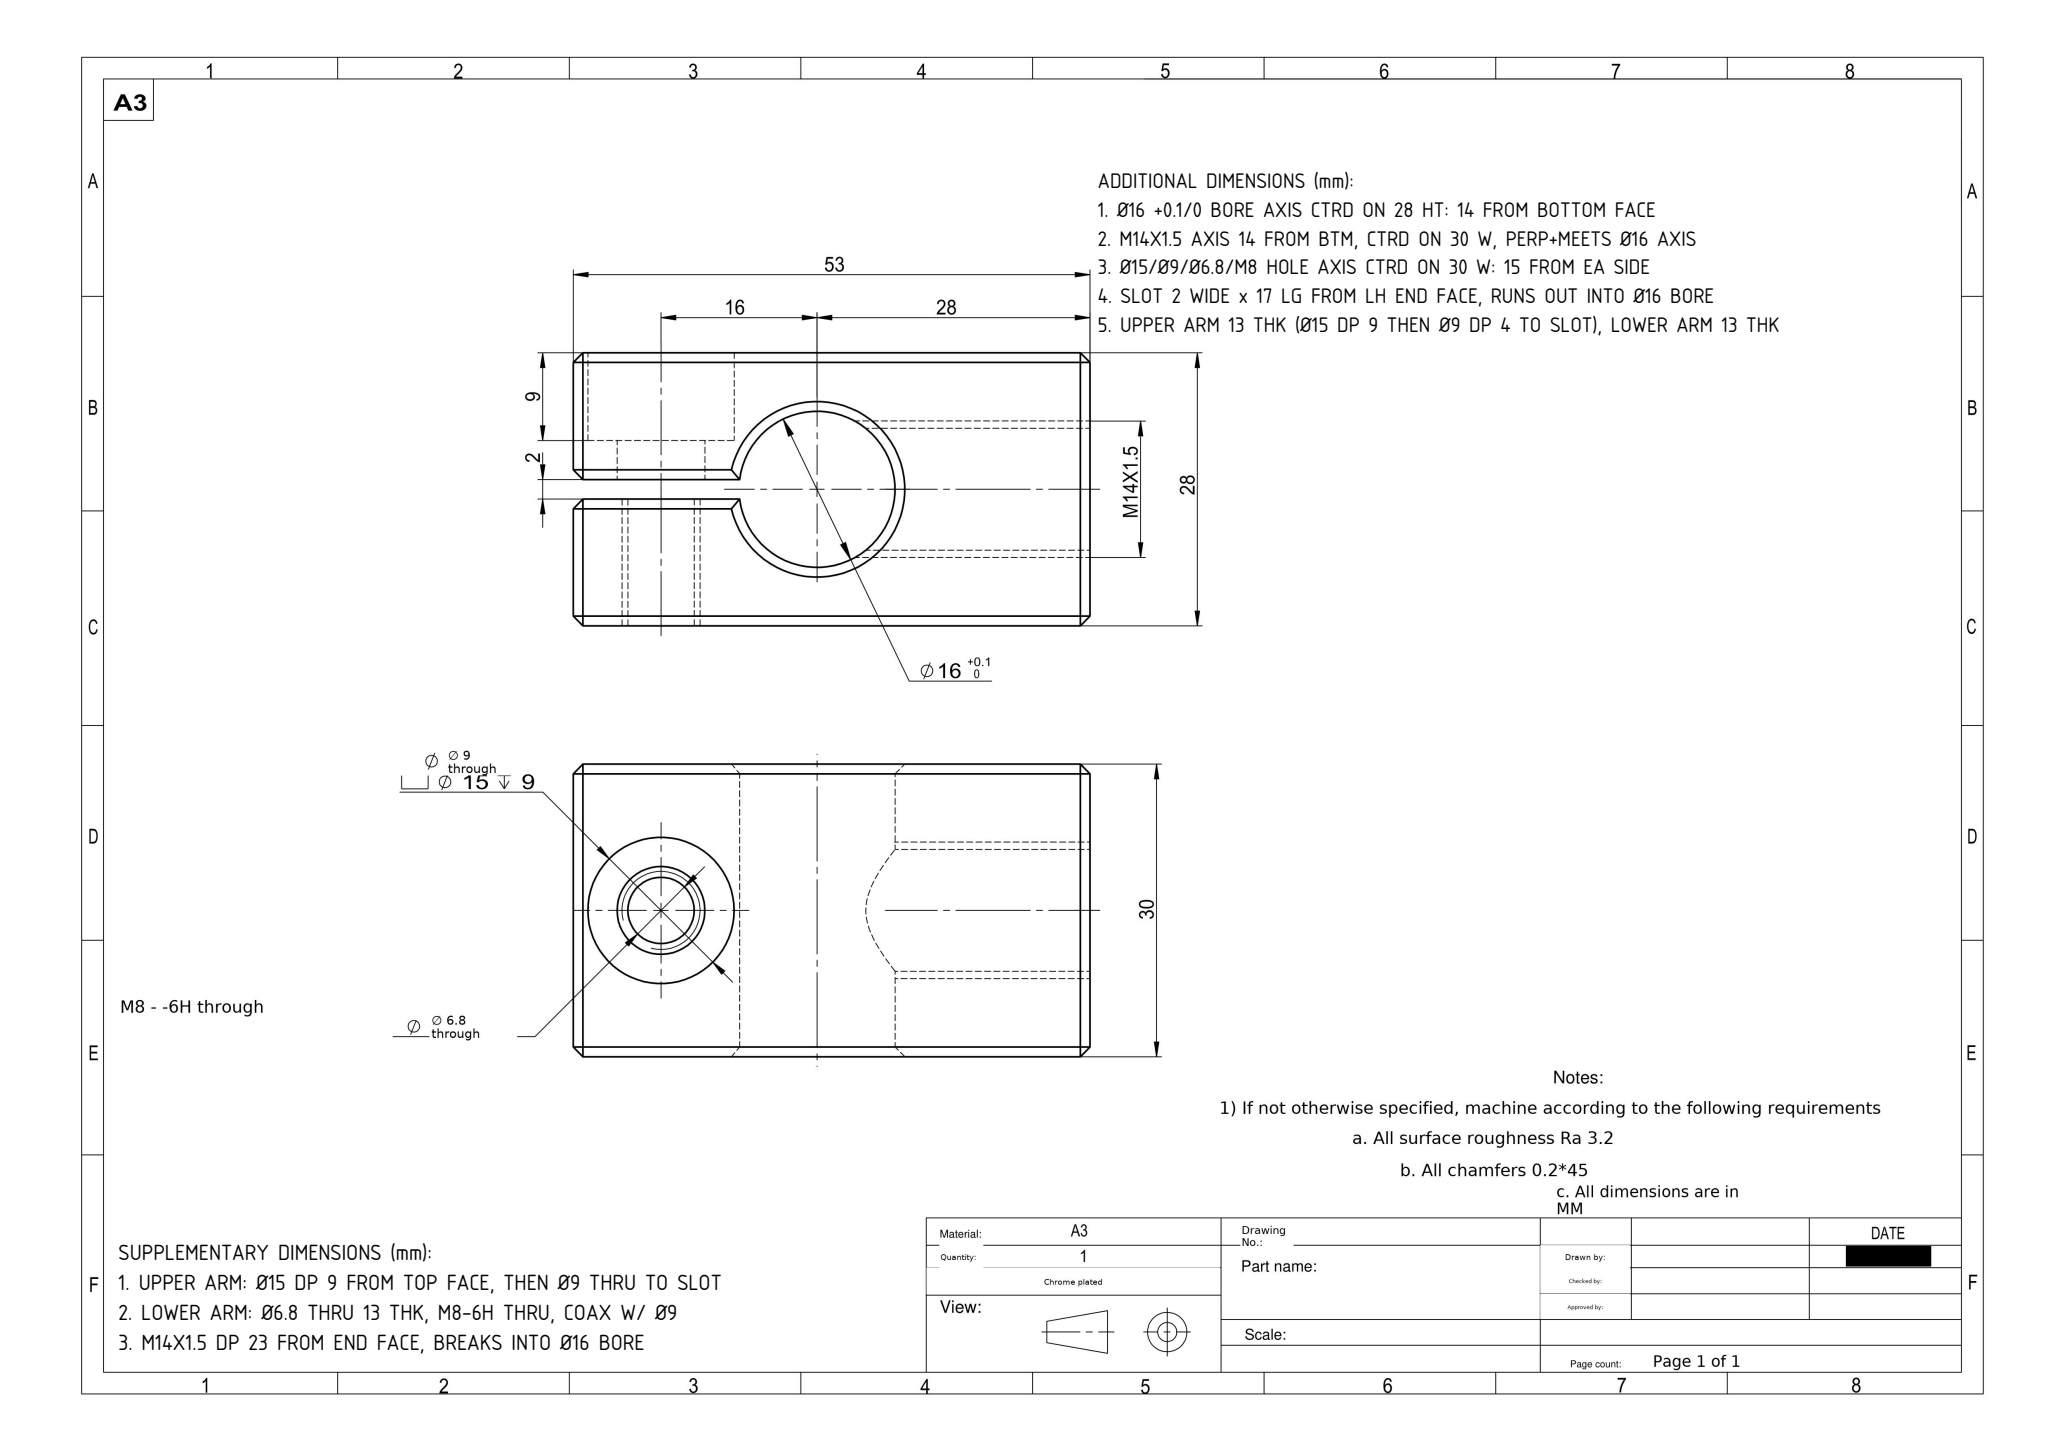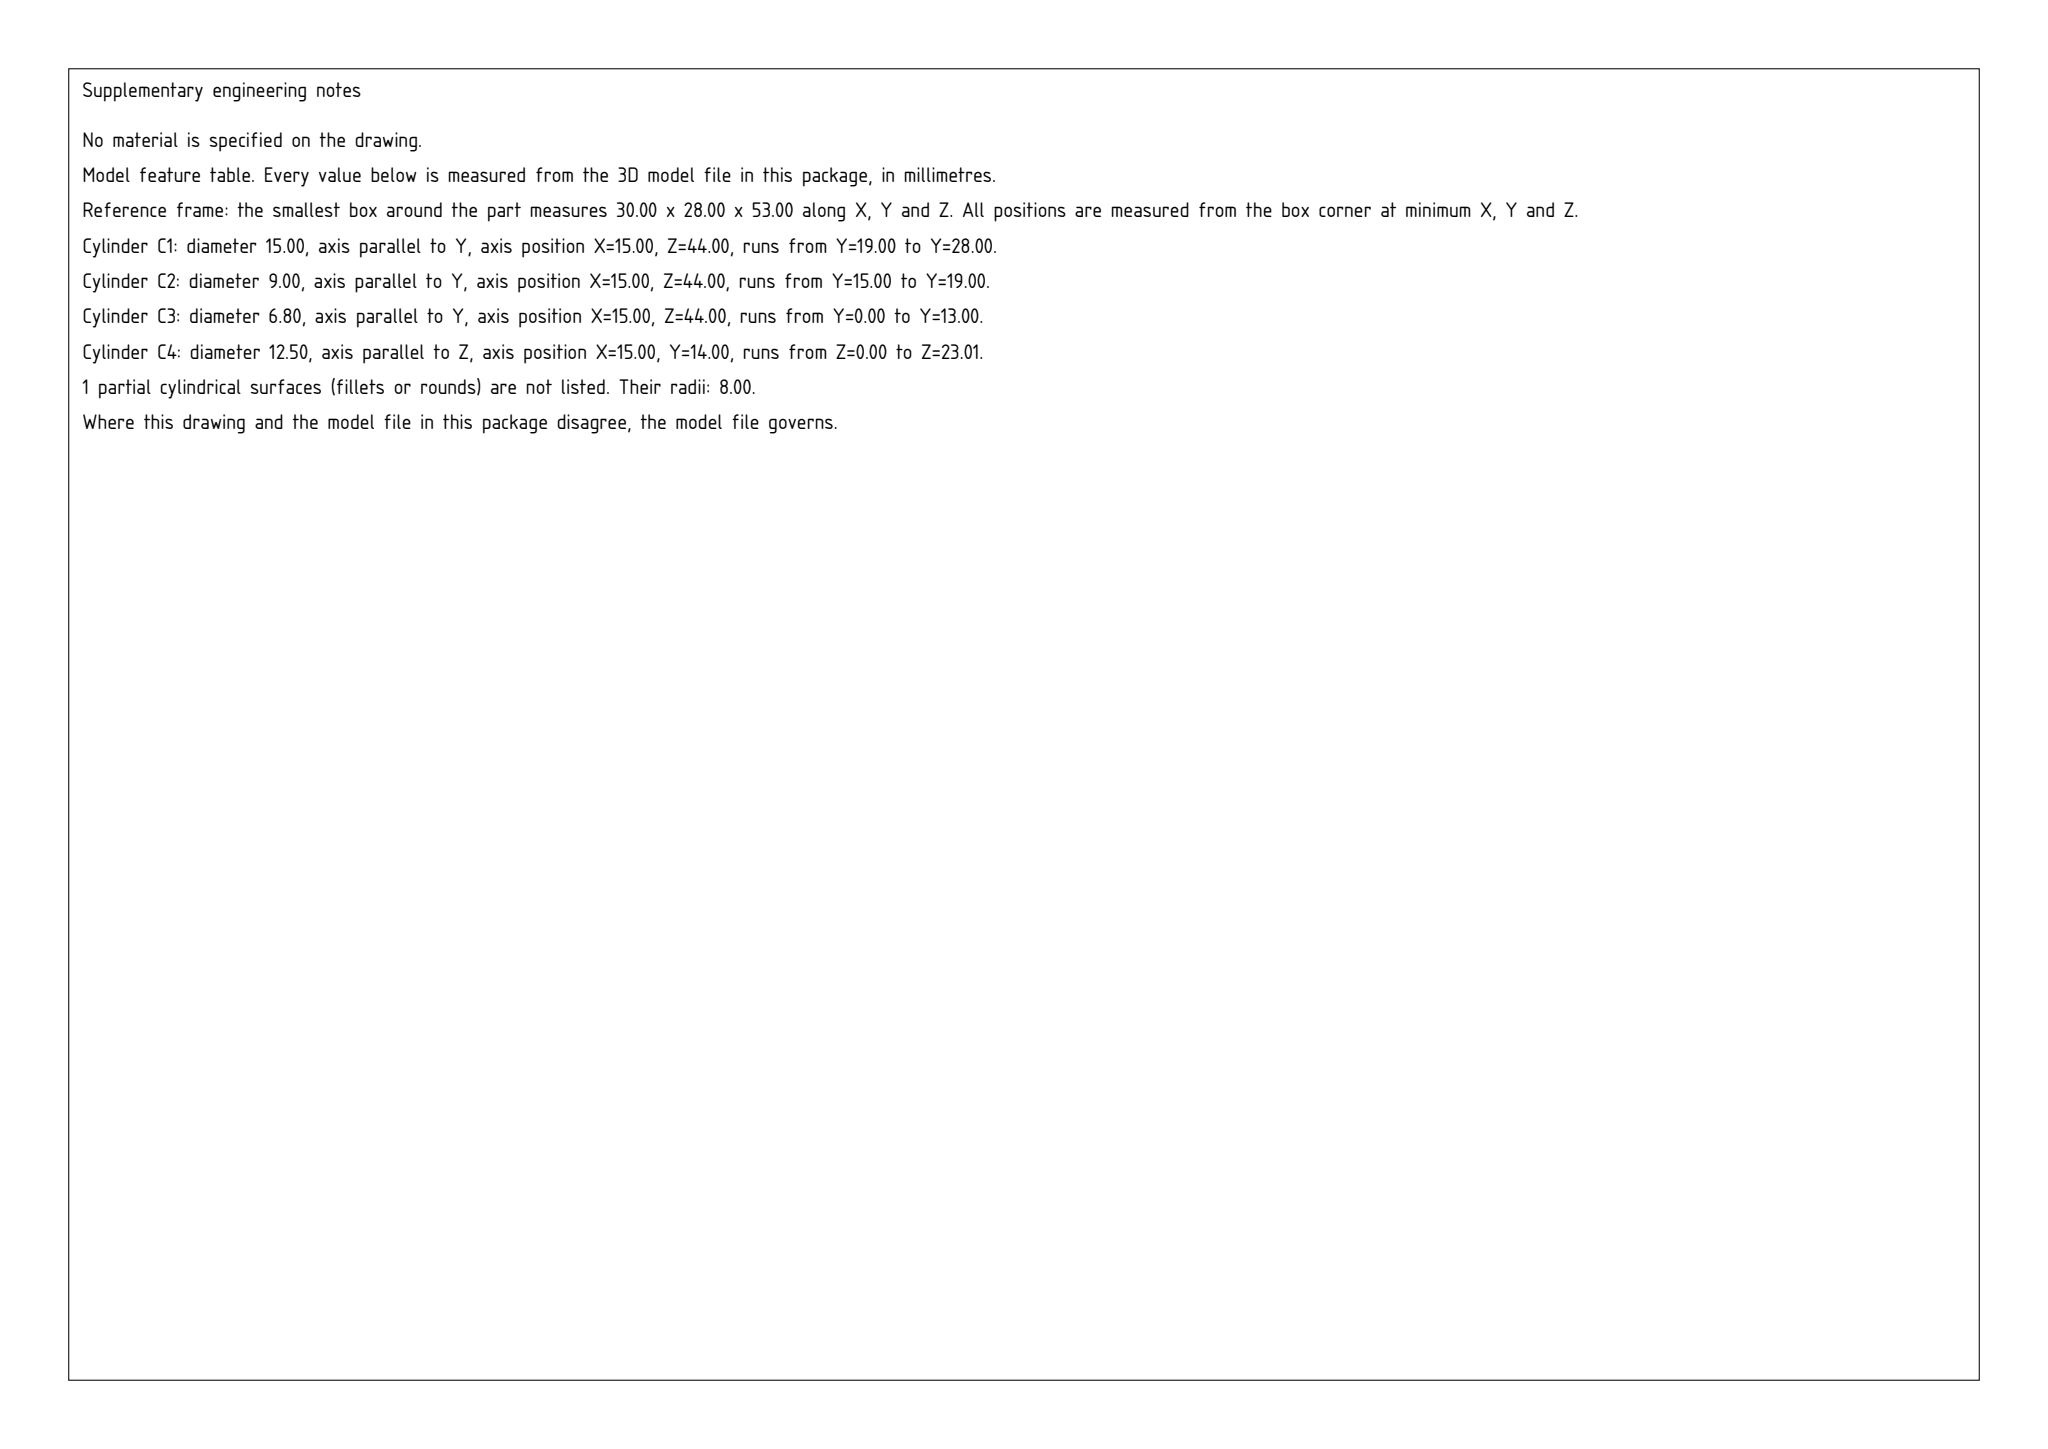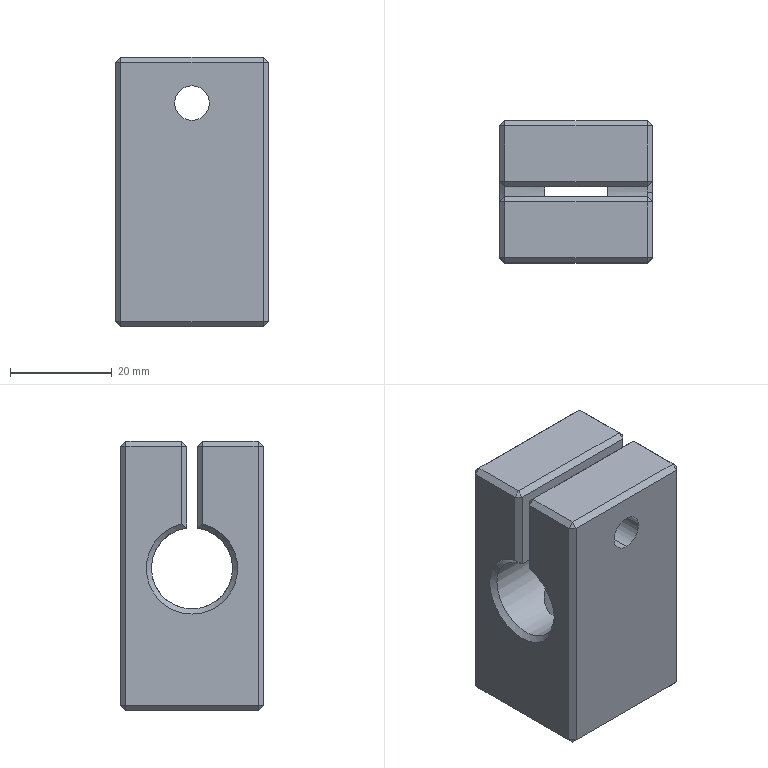Part | SolidWorks | mm | 1 solid | 54 faces | box 30 x 28 x 53 mm | volume 32288 mm3 | plane 42 | cylinder 9 | cone 3 | commonest cylinder face diameters 6.8 x2 15 x2 9 x2 12.5 x2 16 x1
build123d program:
from build123d import *

# Parameters (mm, degrees)
SKETCH1_W                                         = 53
SKETCH1_H                                         = 28
SKETCH1_R                                         = 8
BOSS_EXTRUDE1_DEPTH                               = 15
M14X1_5_TAPPED_HOLE1_REACH                        = 58.833
M14X1_5_TAPPED_HOLE1_BORE_R                       = 6.25
CUT_EXTRUDE1_DEPTH                                = 35.713
CUT_EXTRUDE1_DEPTH_BACK                           = 35.713
SKETCH2_W                                         = 25
SKETCH2_H                                         = 2
HOLE_SIZE_ACCORDING_TO_HEXAGON_SOCKET_D           = 9
HOLE_SIZE_ACCORDING_TO_HEXAGON_SOCKET_DEPTH       = 13
HOLE_SIZE_ACCORDING_TO_HEXAGON_SOCKET_CBORE_D     = 15
HOLE_SIZE_ACCORDING_TO_HEXAGON_SOCKET_CBORE_DEPTH = 9
M8_TAPPED_HOLE1_D                                 = 6.8
CHAMFER1_SIZE                                     = 1


with BuildPart() as part:
    # Sketch1 → Boss-Extrude1 (new, symmetric)
    with BuildSketch(Plane(origin=(0, 0, 0), x_dir=(0, 0, -1), z_dir=(1, 0, 0))):
        with Locations((1.5, 0)):
            Rectangle(SKETCH1_W, SKETCH1_H)
        Circle(SKETCH1_R, mode=Mode.SUBTRACT)
    extrude(amount=BOSS_EXTRUDE1_DEPTH, both=True)

    # M14x1.5 Tapped Hole1 bore → M14x1.5 Tapped Hole1 (cut, up to next)
    with BuildSketch(Plane(origin=(0, 0, -28), x_dir=(-1, 0, 0), z_dir=(0, 0, -1)), mode=Mode.PRIVATE) as m14x1_5_tapped_hole1_sk1:
        Circle(M14X1_5_TAPPED_HOLE1_BORE_R)
    m14x1_5_tapped_hole1_tool1 = extrude(m14x1_5_tapped_hole1_sk1.sketch, amount=-M14X1_5_TAPPED_HOLE1_REACH, mode=Mode.PRIVATE) & part.part
    add(m14x1_5_tapped_hole1_tool1.solids().sort_by_distance((0, 0, -28))[0], mode=Mode.SUBTRACT)

    # Sketch2 → Cut-Extrude1 (cut, two sides: drawn at the far end of the back side and taken through both)
    with BuildSketch(Plane(origin=(0, 0, 0), x_dir=(0, 0, -1), z_dir=(1, 0, 0)).offset(-CUT_EXTRUDE1_DEPTH_BACK)):
        with Locations((-12.5, 0)):
            Rectangle(SKETCH2_W, SKETCH2_H)
    extrude(amount=CUT_EXTRUDE1_DEPTH + CUT_EXTRUDE1_DEPTH_BACK, mode=Mode.SUBTRACT)

    # Hole Size _ according to_ Hexagon Socket
    with Locations(Plane(origin=(0, 14, 0), x_dir=(1, 0, 0), z_dir=(0, 1, 0))):
        with Locations((0, -16)):
            CounterBoreHole(HOLE_SIZE_ACCORDING_TO_HEXAGON_SOCKET_D / 2, HOLE_SIZE_ACCORDING_TO_HEXAGON_SOCKET_CBORE_D / 2, HOLE_SIZE_ACCORDING_TO_HEXAGON_SOCKET_CBORE_DEPTH, depth=HOLE_SIZE_ACCORDING_TO_HEXAGON_SOCKET_DEPTH)

    # M8 Tapped Hole1 (through all)
    with Locations(Plane(origin=(0, -1, 0), x_dir=(1, 0, 0), z_dir=(0, 1, 0))):
        with Locations((0, -16)):
            Hole(M8_TAPPED_HOLE1_D / 2)

    # Chamfer1
    chamfer1_edges = [part.edges().sort_by_distance(p)[0] for p in [
        (15, 0, -28),
        (15, 14, -1.5),
        (15, -7.984, -0.501),
        (-15, -7.984, -0.501),
        (-15, -7.5, 25),
        (15, -7.5, 25),
        (0, -1, 25),
        (-15, 1, 16.469),
        (0, 1, 25),
        (-15, -1, 16.469),
        (15, 1, 16.469),
        (15, -1, 16.469),
        (15, 7.5, 25),
        (-15, 14, -1.5),
        (-15, 0, -28),
        (-15, -14, -1.5),
        (-15, 7.5, 25),
        (15, -14, -1.5),
        (0, 14, 25),
        (0, 14, -28),
        (0, -14, -28),
        (0, -14, 25),
    ]]
    chamfer(chamfer1_edges, length=CHAMFER1_SIZE)


solid = part.part